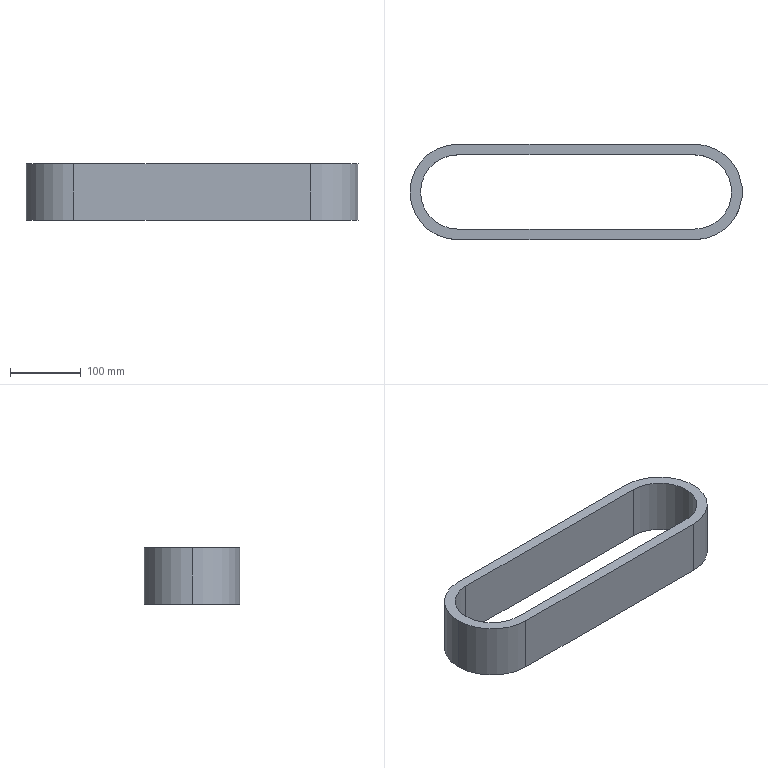Component | SolidWorks | -TractionBelt-2 | 1 solid | 12 faces | box 470 x 135 x 80 mm | volume 1256389 mm3 | cylinder 6 | plane 6 | commonest cylinder face diameters 105 x3 135 x3
build123d program:
from build123d import *

# Parameters (mm, degrees)
BOSS_EXTRUDE1_DEPTH = 40


with BuildPart() as part:
    # Sketch1 → Boss-Extrude1 (new, symmetric)
    with BuildSketch(Plane.XY):
        with BuildLine():
            Line((-95, 67.5), (240, 67.5))
            ThreePointArc((240, 67.5), (307.5, 0), (240, -67.5))
            Line((240, -67.5), (-95, -67.5))
            ThreePointArc((-95, -67.5), (-162.5, 0), (-95, 67.5))
        make_face()
        with BuildLine():
            Line((-95, 52.5), (240, 52.5))
            ThreePointArc((240, 52.5), (292.5, 0), (240, -52.5))
            Line((240, -52.5), (-95, -52.5))
            ThreePointArc((-95, -52.5), (-147.5, 0), (-95, 52.5))
        make_face(mode=Mode.SUBTRACT)
    extrude(amount=BOSS_EXTRUDE1_DEPTH, both=True)


solid = part.part

# Placed as in the assembly
solid = solid.moved(Location((-35, 1239.5, 90), (0, 0, 0)))
STEP:
#1=COLOUR_RGB('',0.7922,0.8196,0.9333);
#2=FILL_AREA_STYLE_COLOUR('',#1);
#3=FILL_AREA_STYLE('',(#2));
#4=SURFACE_STYLE_FILL_AREA(#3);
#5=SURFACE_SIDE_STYLE('',(#4));
#6=SURFACE_STYLE_USAGE(.BOTH.,#5);
#7=PRESENTATION_STYLE_ASSIGNMENT((#6));
#8=CARTESIAN_POINT('',(-5.118,50.866,5.118));
#9=VERTEX_POINT('',#8);
#10=CARTESIAN_POINT('',(-7.185,48.799,5.118));
#11=VERTEX_POINT('',#10);
#12=CARTESIAN_POINT('',(-5.118,48.799,5.118));
#13=DIRECTION('',(0.,0.,1.));
#14=DIRECTION('',(1.,0.,0.));
#15=AXIS2_PLACEMENT_3D('',#12,#13,#14);
#16=CIRCLE('',#15,2.067);
#17=EDGE_CURVE('',#9,#11,#16,.T.);
#18=ORIENTED_EDGE('',*,*,#17,.T.);
#19=CARTESIAN_POINT('',(-7.185,48.799,1.969));
#20=VERTEX_POINT('',#19);
#21=CARTESIAN_POINT('',(-7.185,48.799,5.118));
#22=DIRECTION('',(0.,0.,-1.));
#23=VECTOR('',#22,39.37);
#24=LINE('',#21,#23);
#25=EDGE_CURVE('',#11,#20,#24,.T.);
#26=ORIENTED_EDGE('',*,*,#25,.T.);
#27=CARTESIAN_POINT('',(-5.118,50.866,1.969));
#28=VERTEX_POINT('',#27);
#29=CARTESIAN_POINT('',(-5.118,48.799,1.969));
#30=DIRECTION('',(0.,0.,1.));
#31=DIRECTION('',(1.,0.,0.));
#32=AXIS2_PLACEMENT_3D('',#29,#30,#31);
#33=CIRCLE('',#32,2.067);
#34=EDGE_CURVE('',#28,#20,#33,.T.);
#35=ORIENTED_EDGE('',*,*,#34,.F.);
#36=CARTESIAN_POINT('',(-5.118,50.866,5.118));
#37=DIRECTION('',(0.,0.,-1.));
#38=VECTOR('',#37,39.37);
#39=LINE('',#36,#38);
#40=EDGE_CURVE('',#9,#28,#39,.T.);
#41=ORIENTED_EDGE('',*,*,#40,.F.);
#42=EDGE_LOOP('',(#18,#26,#35,#41));
#43=FACE_OUTER_BOUND('',#42,.T.);
#44=CARTESIAN_POINT('',(-5.118,48.799,5.118));
#45=DIRECTION('',(0.,0.,-1.));
#46=DIRECTION('',(-1.,0.,0.));
#47=AXIS2_PLACEMENT_3D('',#44,#45,#46);
#48=CYLINDRICAL_SURFACE('',#47,2.067);
#49=ADVANCED_FACE('',(#43),#48,.F.);
#50=CARTESIAN_POINT('',(-7.776,48.799,5.118));
#51=VERTEX_POINT('',#50);
#52=CARTESIAN_POINT('',(-5.118,46.142,5.118));
#53=VERTEX_POINT('',#52);
#54=CARTESIAN_POINT('',(-5.118,48.799,5.118));
#55=DIRECTION('',(0.,0.,1.));
#56=DIRECTION('',(1.,0.,0.));
#57=AXIS2_PLACEMENT_3D('',#54,#55,#56);
#58=CIRCLE('',#57,2.657);
#59=EDGE_CURVE('',#51,#53,#58,.T.);
#60=ORIENTED_EDGE('',*,*,#59,.F.);
#61=CARTESIAN_POINT('',(-7.776,48.799,1.969));
#62=VERTEX_POINT('',#61);
#63=CARTESIAN_POINT('',(-7.776,48.799,5.118));
#64=DIRECTION('',(0.,0.,-1.));
#65=VECTOR('',#64,39.37);
#66=LINE('',#63,#65);
#67=EDGE_CURVE('',#51,#62,#66,.T.);
#68=ORIENTED_EDGE('',*,*,#67,.T.);
#69=CARTESIAN_POINT('',(-5.118,46.142,1.969));
#70=VERTEX_POINT('',#69);
#71=CARTESIAN_POINT('',(-5.118,48.799,1.969));
#72=DIRECTION('',(0.,0.,1.));
#73=DIRECTION('',(1.,0.,0.));
#74=AXIS2_PLACEMENT_3D('',#71,#72,#73);
#75=CIRCLE('',#74,2.657);
#76=EDGE_CURVE('',#62,#70,#75,.T.);
#77=ORIENTED_EDGE('',*,*,#76,.T.);
#78=CARTESIAN_POINT('',(-5.118,46.142,5.118));
#79=DIRECTION('',(0.,0.,-1.));
#80=VECTOR('',#79,39.37);
#81=LINE('',#78,#80);
#82=EDGE_CURVE('',#53,#70,#81,.T.);
#83=ORIENTED_EDGE('',*,*,#82,.F.);
#84=EDGE_LOOP('',(#60,#68,#77,#83));
#85=FACE_OUTER_BOUND('',#84,.T.);
#86=CARTESIAN_POINT('',(-5.118,48.799,5.118));
#87=DIRECTION('',(0.,0.,-1.));
#88=DIRECTION('',(-1.,0.,0.));
#89=AXIS2_PLACEMENT_3D('',#86,#87,#88);
#90=CYLINDRICAL_SURFACE('',#89,2.657);
#91=ADVANCED_FACE('',(#85),#90,.T.);
#92=CARTESIAN_POINT('',(-5.118,51.457,5.118));
#93=VERTEX_POINT('',#92);
#94=CARTESIAN_POINT('',(-5.118,48.799,5.118));
#95=DIRECTION('',(0.,0.,1.));
#96=DIRECTION('',(1.,0.,0.));
#97=AXIS2_PLACEMENT_3D('',#94,#95,#96);
#98=CIRCLE('',#97,2.657);
#99=EDGE_CURVE('',#93,#51,#98,.T.);
#100=ORIENTED_EDGE('',*,*,#99,.T.);
#101=ORIENTED_EDGE('',*,*,#59,.T.);
#102=CARTESIAN_POINT('',(8.071,46.142,5.118));
#103=VERTEX_POINT('',#102);
#104=CARTESIAN_POINT('',(-5.118,46.142,5.118));
#105=DIRECTION('',(1.,0.,0.));
#106=VECTOR('',#105,39.37);
#107=LINE('',#104,#106);
#108=EDGE_CURVE('',#53,#103,#107,.T.);
#109=ORIENTED_EDGE('',*,*,#108,.T.);
#110=CARTESIAN_POINT('',(8.071,51.457,5.118));
#111=VERTEX_POINT('',#110);
#112=CARTESIAN_POINT('',(8.071,48.799,5.118));
#113=DIRECTION('',(0.,0.,1.));
#114=DIRECTION('',(1.,0.,0.));
#115=AXIS2_PLACEMENT_3D('',#112,#113,#114);
#116=CIRCLE('',#115,2.657);
#117=EDGE_CURVE('',#103,#111,#116,.T.);
#118=ORIENTED_EDGE('',*,*,#117,.T.);
#119=CARTESIAN_POINT('',(-5.118,51.457,5.118));
#120=DIRECTION('',(-1.,0.,0.));
#121=VECTOR('',#120,39.37);
#122=LINE('',#119,#121);
#123=EDGE_CURVE('',#111,#93,#122,.T.);
#124=ORIENTED_EDGE('',*,*,#123,.T.);
#125=EDGE_LOOP('',(#100,#101,#109,#118,#124));
#126=FACE_OUTER_BOUND('',#125,.T.);
#127=CARTESIAN_POINT('',(-5.118,46.732,5.118));
#128=VERTEX_POINT('',#127);
#129=CARTESIAN_POINT('',(8.071,46.732,5.118));
#130=VERTEX_POINT('',#129);
#131=CARTESIAN_POINT('',(-5.118,46.732,5.118));
#132=DIRECTION('',(1.,0.,0.));
#133=VECTOR('',#132,39.37);
#134=LINE('',#131,#133);
#135=EDGE_CURVE('',#128,#130,#134,.T.);
#136=ORIENTED_EDGE('',*,*,#135,.F.);
#137=CARTESIAN_POINT('',(-5.118,48.799,5.118));
#138=DIRECTION('',(0.,0.,1.));
#139=DIRECTION('',(1.,0.,0.));
#140=AXIS2_PLACEMENT_3D('',#137,#138,#139);
#141=CIRCLE('',#140,2.067);
#142=EDGE_CURVE('',#11,#128,#141,.T.);
#143=ORIENTED_EDGE('',*,*,#142,.F.);
#144=ORIENTED_EDGE('',*,*,#17,.F.);
#145=CARTESIAN_POINT('',(8.071,50.866,5.118));
#146=VERTEX_POINT('',#145);
#147=CARTESIAN_POINT('',(-5.118,50.866,5.118));
#148=DIRECTION('',(-1.,0.,0.));
#149=VECTOR('',#148,39.37);
#150=LINE('',#147,#149);
#151=EDGE_CURVE('',#146,#9,#150,.T.);
#152=ORIENTED_EDGE('',*,*,#151,.F.);
#153=CARTESIAN_POINT('',(8.071,48.799,5.118));
#154=DIRECTION('',(0.,0.,1.));
#155=DIRECTION('',(1.,0.,0.));
#156=AXIS2_PLACEMENT_3D('',#153,#154,#155);
#157=CIRCLE('',#156,2.067);
#158=EDGE_CURVE('',#130,#146,#157,.T.);
#159=ORIENTED_EDGE('',*,*,#158,.F.);
#160=EDGE_LOOP('',(#136,#143,#144,#152,#159));
#161=FACE_BOUND('',#160,.T.);
#162=CARTESIAN_POINT('',(-5.118,48.799,5.118));
#163=DIRECTION('',(0.,0.,1.));
#164=DIRECTION('',(1.,0.,0.));
#165=AXIS2_PLACEMENT_3D('',#162,#163,#164);
#166=PLANE('',#165);
#167=ADVANCED_FACE('',(#126,#161),#166,.T.);
#168=CARTESIAN_POINT('',(-5.118,51.457,1.969));
#169=VERTEX_POINT('',#168);
#170=CARTESIAN_POINT('',(-5.118,48.799,1.969));
#171=DIRECTION('',(0.,0.,1.));
#172=DIRECTION('',(1.,0.,0.));
#173=AXIS2_PLACEMENT_3D('',#170,#171,#172);
#174=CIRCLE('',#173,2.657);
#175=EDGE_CURVE('',#169,#62,#174,.T.);
#176=ORIENTED_EDGE('',*,*,#175,.F.);
#177=CARTESIAN_POINT('',(8.071,51.457,1.969));
#178=VERTEX_POINT('',#177);
#179=CARTESIAN_POINT('',(-5.118,51.457,1.969));
#180=DIRECTION('',(-1.,0.,0.));
#181=VECTOR('',#180,39.37);
#182=LINE('',#179,#181);
#183=EDGE_CURVE('',#178,#169,#182,.T.);
#184=ORIENTED_EDGE('',*,*,#183,.F.);
#185=CARTESIAN_POINT('',(8.071,46.142,1.969));
#186=VERTEX_POINT('',#185);
#187=CARTESIAN_POINT('',(8.071,48.799,1.969));
#188=DIRECTION('',(0.,0.,1.));
#189=DIRECTION('',(1.,0.,0.));
#190=AXIS2_PLACEMENT_3D('',#187,#188,#189);
#191=CIRCLE('',#190,2.657);
#192=EDGE_CURVE('',#186,#178,#191,.T.);
#193=ORIENTED_EDGE('',*,*,#192,.F.);
#194=CARTESIAN_POINT('',(-5.118,46.142,1.969));
#195=DIRECTION('',(1.,0.,0.));
#196=VECTOR('',#195,39.37);
#197=LINE('',#194,#196);
#198=EDGE_CURVE('',#70,#186,#197,.T.);
#199=ORIENTED_EDGE('',*,*,#198,.F.);
#200=ORIENTED_EDGE('',*,*,#76,.F.);
#201=EDGE_LOOP('',(#176,#184,#193,#199,#200));
#202=FACE_OUTER_BOUND('',#201,.T.);
#203=ORIENTED_EDGE('',*,*,#34,.T.);
#204=CARTESIAN_POINT('',(-5.118,46.732,1.969));
#205=VERTEX_POINT('',#204);
#206=CARTESIAN_POINT('',(-5.118,48.799,1.969));
#207=DIRECTION('',(0.,0.,1.));
#208=DIRECTION('',(1.,0.,0.));
#209=AXIS2_PLACEMENT_3D('',#206,#207,#208);
#210=CIRCLE('',#209,2.067);
#211=EDGE_CURVE('',#20,#205,#210,.T.);
#212=ORIENTED_EDGE('',*,*,#211,.T.);
#213=CARTESIAN_POINT('',(8.071,46.732,1.969));
#214=VERTEX_POINT('',#213);
#215=CARTESIAN_POINT('',(-5.118,46.732,1.969));
#216=DIRECTION('',(1.,0.,0.));
#217=VECTOR('',#216,39.37);
#218=LINE('',#215,#217);
#219=EDGE_CURVE('',#205,#214,#218,.T.);
#220=ORIENTED_EDGE('',*,*,#219,.T.);
#221=CARTESIAN_POINT('',(8.071,50.866,1.969));
#222=VERTEX_POINT('',#221);
#223=CARTESIAN_POINT('',(8.071,48.799,1.969));
#224=DIRECTION('',(0.,0.,1.));
#225=DIRECTION('',(1.,0.,0.));
#226=AXIS2_PLACEMENT_3D('',#223,#224,#225);
#227=CIRCLE('',#226,2.067);
#228=EDGE_CURVE('',#214,#222,#227,.T.);
#229=ORIENTED_EDGE('',*,*,#228,.T.);
#230=CARTESIAN_POINT('',(-5.118,50.866,1.969));
#231=DIRECTION('',(-1.,0.,0.));
#232=VECTOR('',#231,39.37);
#233=LINE('',#230,#232);
#234=EDGE_CURVE('',#222,#28,#233,.T.);
#235=ORIENTED_EDGE('',*,*,#234,.T.);
#236=EDGE_LOOP('',(#203,#212,#220,#229,#235));
#237=FACE_BOUND('',#236,.T.);
#238=CARTESIAN_POINT('',(-5.118,48.799,1.969));
#239=DIRECTION('',(0.,0.,1.));
#240=DIRECTION('',(1.,0.,0.));
#241=AXIS2_PLACEMENT_3D('',#238,#239,#240);
#242=PLANE('',#241);
#243=ADVANCED_FACE('',(#202,#237),#242,.F.);
#244=ORIENTED_EDGE('',*,*,#67,.F.);
#245=ORIENTED_EDGE('',*,*,#99,.F.);
#246=CARTESIAN_POINT('',(-5.118,51.457,5.118));
#247=DIRECTION('',(0.,0.,-1.));
#248=VECTOR('',#247,39.37);
#249=LINE('',#246,#248);
#250=EDGE_CURVE('',#93,#169,#249,.T.);
#251=ORIENTED_EDGE('',*,*,#250,.T.);
#252=ORIENTED_EDGE('',*,*,#175,.T.);
#253=EDGE_LOOP('',(#244,#245,#251,#252));
#254=FACE_OUTER_BOUND('',#253,.T.);
#255=CARTESIAN_POINT('',(-5.118,48.799,5.118));
#256=DIRECTION('',(0.,0.,-1.));
#257=DIRECTION('',(-1.,0.,0.));
#258=AXIS2_PLACEMENT_3D('',#255,#256,#257);
#259=CYLINDRICAL_SURFACE('',#258,2.657);
#260=ADVANCED_FACE('',(#254),#259,.T.);
#261=ORIENTED_EDGE('',*,*,#198,.T.);
#262=CARTESIAN_POINT('',(8.071,46.142,5.118));
#263=DIRECTION('',(0.,0.,-1.));
#264=VECTOR('',#263,39.37);
#265=LINE('',#262,#264);
#266=EDGE_CURVE('',#103,#186,#265,.T.);
#267=ORIENTED_EDGE('',*,*,#266,.F.);
#268=ORIENTED_EDGE('',*,*,#108,.F.);
#269=ORIENTED_EDGE('',*,*,#82,.T.);
#270=EDGE_LOOP('',(#261,#267,#268,#269));
#271=FACE_OUTER_BOUND('',#270,.T.);
#272=CARTESIAN_POINT('',(-5.118,46.142,5.118));
#273=DIRECTION('',(0.,1.,0.));
#274=DIRECTION('',(0.,0.,1.));
#275=AXIS2_PLACEMENT_3D('',#272,#273,#274);
#276=PLANE('',#275);
#277=ADVANCED_FACE('',(#271),#276,.F.);
#278=ORIENTED_EDGE('',*,*,#192,.T.);
#279=CARTESIAN_POINT('',(8.071,51.457,5.118));
#280=DIRECTION('',(0.,0.,-1.));
#281=VECTOR('',#280,39.37);
#282=LINE('',#279,#281);
#283=EDGE_CURVE('',#111,#178,#282,.T.);
#284=ORIENTED_EDGE('',*,*,#283,.F.);
#285=ORIENTED_EDGE('',*,*,#117,.F.);
#286=ORIENTED_EDGE('',*,*,#266,.T.);
#287=EDGE_LOOP('',(#278,#284,#285,#286));
#288=FACE_OUTER_BOUND('',#287,.T.);
#289=CARTESIAN_POINT('',(8.071,48.799,5.118));
#290=DIRECTION('',(0.,0.,-1.));
#291=DIRECTION('',(-1.,0.,0.));
#292=AXIS2_PLACEMENT_3D('',#289,#290,#291);
#293=CYLINDRICAL_SURFACE('',#292,2.657);
#294=ADVANCED_FACE('',(#288),#293,.T.);
#295=ORIENTED_EDGE('',*,*,#183,.T.);
#296=ORIENTED_EDGE('',*,*,#250,.F.);
#297=ORIENTED_EDGE('',*,*,#123,.F.);
#298=ORIENTED_EDGE('',*,*,#283,.T.);
#299=EDGE_LOOP('',(#295,#296,#297,#298));
#300=FACE_OUTER_BOUND('',#299,.T.);
#301=CARTESIAN_POINT('',(-5.118,51.457,5.118));
#302=DIRECTION('',(0.,-1.,0.));
#303=DIRECTION('',(0.,0.,-1.));
#304=AXIS2_PLACEMENT_3D('',#301,#302,#303);
#305=PLANE('',#304);
#306=ADVANCED_FACE('',(#300),#305,.F.);
#307=ORIENTED_EDGE('',*,*,#25,.F.);
#308=ORIENTED_EDGE('',*,*,#142,.T.);
#309=CARTESIAN_POINT('',(-5.118,46.732,5.118));
#310=DIRECTION('',(0.,0.,-1.));
#311=VECTOR('',#310,39.37);
#312=LINE('',#309,#311);
#313=EDGE_CURVE('',#128,#205,#312,.T.);
#314=ORIENTED_EDGE('',*,*,#313,.T.);
#315=ORIENTED_EDGE('',*,*,#211,.F.);
#316=EDGE_LOOP('',(#307,#308,#314,#315));
#317=FACE_OUTER_BOUND('',#316,.T.);
#318=CARTESIAN_POINT('',(-5.118,48.799,5.118));
#319=DIRECTION('',(0.,0.,-1.));
#320=DIRECTION('',(-1.,0.,0.));
#321=AXIS2_PLACEMENT_3D('',#318,#319,#320);
#322=CYLINDRICAL_SURFACE('',#321,2.067);
#323=ADVANCED_FACE('',(#317),#322,.F.);
#324=ORIENTED_EDGE('',*,*,#219,.F.);
#325=ORIENTED_EDGE('',*,*,#313,.F.);
#326=ORIENTED_EDGE('',*,*,#135,.T.);
#327=CARTESIAN_POINT('',(8.071,46.732,5.118));
#328=DIRECTION('',(0.,0.,-1.));
#329=VECTOR('',#328,39.37);
#330=LINE('',#327,#329);
#331=EDGE_CURVE('',#130,#214,#330,.T.);
#332=ORIENTED_EDGE('',*,*,#331,.T.);
#333=EDGE_LOOP('',(#324,#325,#326,#332));
#334=FACE_OUTER_BOUND('',#333,.T.);
#335=CARTESIAN_POINT('',(-5.118,46.732,5.118));
#336=DIRECTION('',(0.,1.,0.));
#337=DIRECTION('',(0.,0.,1.));
#338=AXIS2_PLACEMENT_3D('',#335,#336,#337);
#339=PLANE('',#338);
#340=ADVANCED_FACE('',(#334),#339,.T.);
#341=ORIENTED_EDGE('',*,*,#228,.F.);
#342=ORIENTED_EDGE('',*,*,#331,.F.);
#343=ORIENTED_EDGE('',*,*,#158,.T.);
#344=CARTESIAN_POINT('',(8.071,50.866,5.118));
#345=DIRECTION('',(0.,0.,-1.));
#346=VECTOR('',#345,39.37);
#347=LINE('',#344,#346);
#348=EDGE_CURVE('',#146,#222,#347,.T.);
#349=ORIENTED_EDGE('',*,*,#348,.T.);
#350=EDGE_LOOP('',(#341,#342,#343,#349));
#351=FACE_OUTER_BOUND('',#350,.T.);
#352=CARTESIAN_POINT('',(8.071,48.799,5.118));
#353=DIRECTION('',(0.,0.,-1.));
#354=DIRECTION('',(-1.,0.,0.));
#355=AXIS2_PLACEMENT_3D('',#352,#353,#354);
#356=CYLINDRICAL_SURFACE('',#355,2.067);
#357=ADVANCED_FACE('',(#351),#356,.F.);
#358=ORIENTED_EDGE('',*,*,#234,.F.);
#359=ORIENTED_EDGE('',*,*,#348,.F.);
#360=ORIENTED_EDGE('',*,*,#151,.T.);
#361=ORIENTED_EDGE('',*,*,#40,.T.);
#362=EDGE_LOOP('',(#358,#359,#360,#361));
#363=FACE_OUTER_BOUND('',#362,.T.);
#364=CARTESIAN_POINT('',(-5.118,50.866,5.118));
#365=DIRECTION('',(0.,-1.,0.));
#366=DIRECTION('',(0.,0.,-1.));
#367=AXIS2_PLACEMENT_3D('',#364,#365,#366);
#368=PLANE('',#367);
#369=ADVANCED_FACE('',(#363),#368,.T.);
#370=CLOSED_SHELL('',(#49,#91,#167,#243,#260,#277,#294,#306,#323,#340,#357,#369));
#371=MANIFOLD_SOLID_BREP('',#370);
#372=STYLED_ITEM('',(#7),#371);
#373=(LENGTH_UNIT()NAMED_UNIT(*)SI_UNIT($,.METRE.));
#374=LENGTH_MEASURE_WITH_UNIT(LENGTH_MEASURE(0.0254),#373);
#375=DIMENSIONAL_EXPONENTS(1.,0.,0.,0.,0.,0.,0.);
#376=(CONVERSION_BASED_UNIT('',#374)LENGTH_UNIT()NAMED_UNIT(#375));
#377=UNCERTAINTY_MEASURE_WITH_UNIT(LENGTH_MEASURE(0.00001),#376,'','');
#378=(NAMED_UNIT(*)PLANE_ANGLE_UNIT()SI_UNIT($,.RADIAN.));
#379=(NAMED_UNIT(*)SI_UNIT($,.STERADIAN.)SOLID_ANGLE_UNIT());
#380=(GEOMETRIC_REPRESENTATION_CONTEXT(3)GLOBAL_UNCERTAINTY_ASSIGNED_CONTEXT((#377))GLOBAL_UNIT_ASSIGNED_CONTEXT((#376,#378,#379))REPRESENTATION_CONTEXT('',''));
#381=MECHANICAL_DESIGN_GEOMETRIC_PRESENTATION_REPRESENTATION('',(#372),#380);
#382=CARTESIAN_POINT('',(0.,0.,0.));
#383=DIRECTION('',(0.,0.,1.));
#384=DIRECTION('',(1.,0.,0.));
#385=AXIS2_PLACEMENT_3D('',#382,#383,#384);
#386=(LENGTH_UNIT()NAMED_UNIT(*)SI_UNIT($,.METRE.));
#387=LENGTH_MEASURE_WITH_UNIT(LENGTH_MEASURE(0.0254),#386);
#388=DIMENSIONAL_EXPONENTS(1.,0.,0.,0.,0.,0.,0.);
#389=(CONVERSION_BASED_UNIT('',#387)LENGTH_UNIT()NAMED_UNIT(#388));
#390=UNCERTAINTY_MEASURE_WITH_UNIT(LENGTH_MEASURE(0.00001),#389,'','');
#391=(NAMED_UNIT(*)PLANE_ANGLE_UNIT()SI_UNIT($,.RADIAN.));
#392=(NAMED_UNIT(*)SI_UNIT($,.STERADIAN.)SOLID_ANGLE_UNIT());
#393=(GEOMETRIC_REPRESENTATION_CONTEXT(3)GLOBAL_UNCERTAINTY_ASSIGNED_CONTEXT((#390))GLOBAL_UNIT_ASSIGNED_CONTEXT((#389,#391,#392))REPRESENTATION_CONTEXT('',''));
#394=ADVANCED_BREP_SHAPE_REPRESENTATION('',(#371,#385),#393);
#395=PRESENTATION_LAYER_ASSIGNMENT('','',(#372));